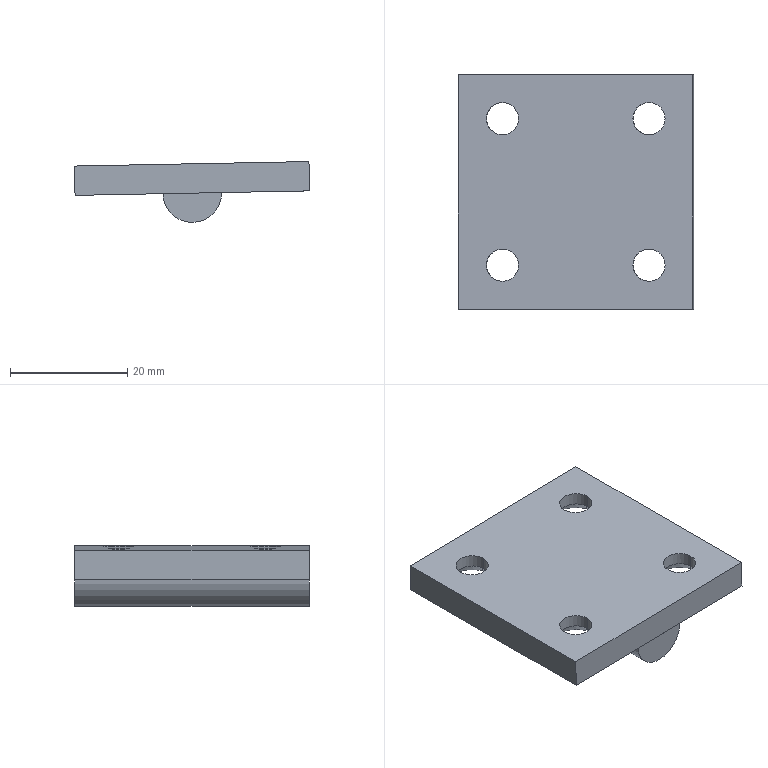Component | SolidWorks | 40X40AluminumAlloyHinge-4 | 2 solids | 27 faces | box 40.09 x 40 x 10.38 mm | volume 8718 mm3 | cylinder 10 | plane 9 | cone 8 | commonest cylinder face diameters 5.5 x8 10 x2 | material A3 Steel
build123d program:
from build123d import *

# Parameters (mm, degrees)
SKETCH1_W                                  = 40
SKETCH1_H                                  = 40
BOSS_EXTRUDE1_DEPTH                        = 5
BOSS_EXTRUDE2_DEPTH                        = 40
HOLE_SIZE_ACCORDING_TO_TYPE_1_OF_S_2_COUNT = 2
HOLE_SIZE_ACCORDING_TO_TYPE_1_OF_S_2_PITCH = 25
HOLE_SIZE_ACCORDING_TO_TYPE_1_OF_S_3_COUNT = 2
HOLE_SIZE_ACCORDING_TO_TYPE_1_OF_S_3_PITCH = 25
HOLE_SIZE_ACCORDING_TO_TYPE_1_OF_S_4_COUNT = 2
HOLE_SIZE_ACCORDING_TO_TYPE_1_OF_S_4_PITCH = 35.355


with BuildPart() as part:
    # Sketch1 → Boss-Extrude1 (new body)
    with BuildSketch(Plane.XY):
        Rectangle(SKETCH1_W, SKETCH1_H)
    extrude(amount=BOSS_EXTRUDE1_DEPTH)

    # Sketch5 → Hole Size _According to_ Type 1 of Slott (revolve, cut)
    with BuildSketch(Plane(origin=(-12.5, 12.5, 5), x_dir=(0, -1, 0), z_dir=(1, 0, 0))):
        Polygon((0, 0), (0, 5), (2.75, 5), (2.75, 2.85), (5.6, 0), align=None)
    hole_size_according_to_type_1_of_slott = revolve(axis=Axis((-12.5, 12.5, 11.35), (0, 0, -1)), mode=Mode.SUBTRACT)

    # Hole Size _According to_ Type 1 of S 2: Hole Size _According to_ Type 1 of Slott ×2
    with Locations(*[(0, -i * HOLE_SIZE_ACCORDING_TO_TYPE_1_OF_S_2_PITCH, 0) for i in range(1, HOLE_SIZE_ACCORDING_TO_TYPE_1_OF_S_2_COUNT)]):
        add(hole_size_according_to_type_1_of_slott, mode=Mode.SUBTRACT)

    # Hole Size _According to_ Type 1 of S 3: Hole Size _According to_ Type 1 of Slott ×2
    with Locations(*[(i * HOLE_SIZE_ACCORDING_TO_TYPE_1_OF_S_3_PITCH, 0, 0) for i in range(1, HOLE_SIZE_ACCORDING_TO_TYPE_1_OF_S_3_COUNT)]):
        add(hole_size_according_to_type_1_of_slott, mode=Mode.SUBTRACT)

    # Hole Size _According to_ Type 1 of S 4: Hole Size _According to_ Type 1 of Slott ×2
    with Locations(*[Vector(0.7071, -0.7071, 0) * (i * HOLE_SIZE_ACCORDING_TO_TYPE_1_OF_S_4_PITCH) for i in range(1, HOLE_SIZE_ACCORDING_TO_TYPE_1_OF_S_4_COUNT)]):
        add(hole_size_according_to_type_1_of_slott, mode=Mode.SUBTRACT)


with BuildPart() as body_2:
    # Sketch2 → Boss-Extrude2 (new body)
    with BuildSketch(Plane(origin=(0, 20, 0), x_dir=(1, 0, 0), z_dir=(0, 1, 0))):
        with BuildLine():
            Line((-5, -5), (5, -5))
            ThreePointArc((5, -5), (0, -10), (-5, -5))
        make_face()
    extrude(amount=-BOSS_EXTRUDE2_DEPTH)


solid = Compound([part.part, body_2.part])

# Placed as in the assembly
solid = solid.moved(Location((-505.846, -2233.022, 1470.376), (-180, 1.091, 0)))
STEP:
#1=COLOUR_RGB('',0.7922,0.8196,0.9333);
#2=FILL_AREA_STYLE_COLOUR('',#1);
#3=FILL_AREA_STYLE('',(#2));
#4=SURFACE_STYLE_FILL_AREA(#3);
#5=SURFACE_SIDE_STYLE('',(#4));
#6=SURFACE_STYLE_USAGE(.BOTH.,#5);
#7=PRESENTATION_STYLE_ASSIGNMENT((#6));
#8=CARTESIAN_POINT('',(-19.908,-87.127,57.495));
#9=VERTEX_POINT('',#8);
#10=CARTESIAN_POINT('',(-20.108,-87.127,57.688));
#11=VERTEX_POINT('',#10);
#12=CARTESIAN_POINT('',(-19.911,-87.127,57.692));
#13=DIRECTION('',(-0.,1.,-0.));
#14=DIRECTION('',(0.01904,0.,-0.9998));
#15=AXIS2_PLACEMENT_3D('',#12,#13,#14);
#16=CIRCLE('',#15,0.1969);
#17=EDGE_CURVE('',#9,#11,#16,.T.);
#18=ORIENTED_EDGE('',*,*,#17,.F.);
#19=CARTESIAN_POINT('',(-19.908,-88.702,57.495));
#20=VERTEX_POINT('',#19);
#21=CARTESIAN_POINT('',(-19.908,-86.687,57.495));
#22=DIRECTION('',(0.,-1.,0.));
#23=VECTOR('',#22,39.37);
#24=LINE('',#21,#23);
#25=EDGE_CURVE('',#9,#20,#24,.T.);
#26=ORIENTED_EDGE('',*,*,#25,.T.);
#27=CARTESIAN_POINT('',(-20.108,-88.702,57.688));
#28=VERTEX_POINT('',#27);
#29=CARTESIAN_POINT('',(-19.911,-88.702,57.692));
#30=DIRECTION('',(0.,-1.,0.));
#31=DIRECTION('',(0.01904,0.,-0.9998));
#32=AXIS2_PLACEMENT_3D('',#29,#30,#31);
#33=CIRCLE('',#32,0.1969);
#34=EDGE_CURVE('',#28,#20,#33,.T.);
#35=ORIENTED_EDGE('',*,*,#34,.F.);
#36=CARTESIAN_POINT('',(-20.108,-86.687,57.688));
#37=DIRECTION('',(0.,-1.,0.));
#38=VECTOR('',#37,39.37);
#39=LINE('',#36,#38);
#40=EDGE_CURVE('',#11,#28,#39,.T.);
#41=ORIENTED_EDGE('',*,*,#40,.F.);
#42=EDGE_LOOP('',(#18,#26,#35,#41));
#43=FACE_OUTER_BOUND('',#42,.T.);
#44=CARTESIAN_POINT('',(-19.911,-86.687,57.692));
#45=DIRECTION('',(0.,-1.,0.));
#46=DIRECTION('',(0.01904,0.,-0.9998));
#47=AXIS2_PLACEMENT_3D('',#44,#45,#46);
#48=CYLINDRICAL_SURFACE('',#47,0.1969);
#49=ADVANCED_FACE('',(#43),#48,.T.);
#50=ORIENTED_EDGE('',*,*,#25,.F.);
#51=CARTESIAN_POINT('',(-19.715,-87.127,57.696));
#52=VERTEX_POINT('',#51);
#53=CARTESIAN_POINT('',(-19.911,-87.127,57.692));
#54=DIRECTION('',(-0.,1.,-0.));
#55=DIRECTION('',(0.01904,0.,-0.9998));
#56=AXIS2_PLACEMENT_3D('',#53,#54,#55);
#57=CIRCLE('',#56,0.1969);
#58=EDGE_CURVE('',#52,#9,#57,.T.);
#59=ORIENTED_EDGE('',*,*,#58,.F.);
#60=CARTESIAN_POINT('',(-19.715,-88.702,57.696));
#61=VERTEX_POINT('',#60);
#62=CARTESIAN_POINT('',(-19.715,-86.687,57.696));
#63=DIRECTION('',(0.,-1.,0.));
#64=VECTOR('',#63,39.37);
#65=LINE('',#62,#64);
#66=EDGE_CURVE('',#52,#61,#65,.T.);
#67=ORIENTED_EDGE('',*,*,#66,.T.);
#68=CARTESIAN_POINT('',(-19.911,-88.702,57.692));
#69=DIRECTION('',(0.,-1.,0.));
#70=DIRECTION('',(0.01904,0.,-0.9998));
#71=AXIS2_PLACEMENT_3D('',#68,#69,#70);
#72=CIRCLE('',#71,0.1969);
#73=EDGE_CURVE('',#20,#61,#72,.T.);
#74=ORIENTED_EDGE('',*,*,#73,.F.);
#75=EDGE_LOOP('',(#50,#59,#67,#74));
#76=FACE_OUTER_BOUND('',#75,.T.);
#77=CARTESIAN_POINT('',(-19.911,-86.687,57.692));
#78=DIRECTION('',(0.,-1.,0.));
#79=DIRECTION('',(0.01904,0.,-0.9998));
#80=AXIS2_PLACEMENT_3D('',#77,#78,#79);
#81=CYLINDRICAL_SURFACE('',#80,0.1969);
#82=ADVANCED_FACE('',(#76),#81,.T.);
#83=CARTESIAN_POINT('',(-20.108,-87.127,57.688));
#84=DIRECTION('',(0.9998,0.,0.01904));
#85=VECTOR('',#84,39.37);
#86=LINE('',#83,#85);
#87=EDGE_CURVE('',#11,#52,#86,.T.);
#88=ORIENTED_EDGE('',*,*,#87,.F.);
#89=ORIENTED_EDGE('',*,*,#40,.T.);
#90=CARTESIAN_POINT('',(-20.108,-88.702,57.688));
#91=DIRECTION('',(-0.9998,-0.,-0.01904));
#92=VECTOR('',#91,39.37);
#93=LINE('',#90,#92);
#94=EDGE_CURVE('',#61,#28,#93,.T.);
#95=ORIENTED_EDGE('',*,*,#94,.F.);
#96=ORIENTED_EDGE('',*,*,#66,.F.);
#97=EDGE_LOOP('',(#88,#89,#95,#96));
#98=FACE_OUTER_BOUND('',#97,.T.);
#99=CARTESIAN_POINT('',(-20.108,-86.687,57.688));
#100=DIRECTION('',(-0.01904,0.,0.9998));
#101=DIRECTION('',(-0.9998,-0.,-0.01904));
#102=AXIS2_PLACEMENT_3D('',#99,#100,#101);
#103=PLANE('',#102);
#104=ADVANCED_FACE('',(#98),#103,.T.);
#105=ORIENTED_EDGE('',*,*,#34,.T.);
#106=ORIENTED_EDGE('',*,*,#73,.T.);
#107=ORIENTED_EDGE('',*,*,#94,.T.);
#108=EDGE_LOOP('',(#105,#106,#107));
#109=FACE_OUTER_BOUND('',#108,.T.);
#110=CARTESIAN_POINT('',(-19.911,-88.702,57.692));
#111=DIRECTION('',(0.,-1.,0.));
#112=DIRECTION('',(0.01904,-0.,-0.9998));
#113=AXIS2_PLACEMENT_3D('',#110,#111,#112);
#114=PLANE('',#113);
#115=ADVANCED_FACE('',(#109),#114,.T.);
#116=ORIENTED_EDGE('',*,*,#58,.T.);
#117=ORIENTED_EDGE('',*,*,#17,.T.);
#118=ORIENTED_EDGE('',*,*,#87,.T.);
#119=EDGE_LOOP('',(#116,#117,#118));
#120=FACE_OUTER_BOUND('',#119,.T.);
#121=CARTESIAN_POINT('',(-20.699,-87.127,57.677));
#122=DIRECTION('',(0.,-1.,0.));
#123=DIRECTION('',(0.01904,-0.,-0.9998));
#124=AXIS2_PLACEMENT_3D('',#121,#122,#123);
#125=PLANE('',#124);
#126=ADVANCED_FACE('',(#120),#125,.F.);
#127=CLOSED_SHELL('',(#49,#82,#104,#115,#126));
#128=MANIFOLD_SOLID_BREP('',#127);
#129=STYLED_ITEM('',(#7),#128);
#130=(LENGTH_UNIT()NAMED_UNIT(*)SI_UNIT($,.METRE.));
#131=LENGTH_MEASURE_WITH_UNIT(LENGTH_MEASURE(0.0254),#130);
#132=DIMENSIONAL_EXPONENTS(1.,0.,0.,0.,0.,0.,0.);
#133=(CONVERSION_BASED_UNIT('',#131)LENGTH_UNIT()NAMED_UNIT(#132));
#134=UNCERTAINTY_MEASURE_WITH_UNIT(LENGTH_MEASURE(0.00001),#133,'','');
#135=(NAMED_UNIT(*)PLANE_ANGLE_UNIT()SI_UNIT($,.RADIAN.));
#136=(NAMED_UNIT(*)SI_UNIT($,.STERADIAN.)SOLID_ANGLE_UNIT());
#137=(GEOMETRIC_REPRESENTATION_CONTEXT(3)GLOBAL_UNCERTAINTY_ASSIGNED_CONTEXT((#134))GLOBAL_UNIT_ASSIGNED_CONTEXT((#133,#135,#136))REPRESENTATION_CONTEXT('',''));
#138=MECHANICAL_DESIGN_GEOMETRIC_PRESENTATION_REPRESENTATION('',(#129),#137);
#139=COLOUR_RGB('',0.7922,0.8196,0.9333);
#140=FILL_AREA_STYLE_COLOUR('',#139);
#141=FILL_AREA_STYLE('',(#140));
#142=SURFACE_STYLE_FILL_AREA(#141);
#143=SURFACE_SIDE_STYLE('',(#142));
#144=SURFACE_STYLE_USAGE(.BOTH.,#143);
#145=PRESENTATION_STYLE_ASSIGNMENT((#144));
#146=CARTESIAN_POINT('',(-20.514,-88.406,57.793));
#147=VERTEX_POINT('',#146);
#148=CARTESIAN_POINT('',(-20.297,-88.406,57.797));
#149=VERTEX_POINT('',#148);
#150=CARTESIAN_POINT('',(-20.406,-88.406,57.795));
#151=DIRECTION('',(0.01904,-0.,-0.9998));
#152=DIRECTION('',(0.9998,0.,0.01904));
#153=AXIS2_PLACEMENT_3D('',#150,#151,#152);
#154=CIRCLE('',#153,0.1083);
#155=EDGE_CURVE('',#147,#149,#154,.T.);
#156=ORIENTED_EDGE('',*,*,#155,.F.);
#157=CARTESIAN_POINT('',(-20.624,-88.406,57.678));
#158=VERTEX_POINT('',#157);
#159=CARTESIAN_POINT('',(-20.624,-88.406,57.678));
#160=DIRECTION('',(-0.6935,-0.,-0.7204));
#161=VECTOR('',#160,39.37);
#162=LINE('',#159,#161);
#163=EDGE_CURVE('',#147,#158,#162,.T.);
#164=ORIENTED_EDGE('',*,*,#163,.T.);
#165=CARTESIAN_POINT('',(-20.183,-88.406,57.687));
#166=VERTEX_POINT('',#165);
#167=CARTESIAN_POINT('',(-20.404,-88.406,57.683));
#168=DIRECTION('',(0.01904,-0.,-0.9998));
#169=DIRECTION('',(0.9998,0.,0.01904));
#170=AXIS2_PLACEMENT_3D('',#167,#168,#169);
#171=CIRCLE('',#170,0.2205);
#172=EDGE_CURVE('',#158,#166,#171,.T.);
#173=ORIENTED_EDGE('',*,*,#172,.T.);
#174=CARTESIAN_POINT('',(-20.183,-88.406,57.687));
#175=DIRECTION('',(0.7204,0.,-0.6935));
#176=VECTOR('',#175,39.37);
#177=LINE('',#174,#176);
#178=EDGE_CURVE('',#149,#166,#177,.T.);
#179=ORIENTED_EDGE('',*,*,#178,.F.);
#180=EDGE_LOOP('',(#156,#164,#173,#179));
#181=FACE_OUTER_BOUND('',#180,.T.);
#182=CARTESIAN_POINT('',(-20.404,-88.406,57.683));
#183=DIRECTION('',(0.01904,-0.,-0.9998));
#184=DIRECTION('',(0.9998,0.,0.01904));
#185=AXIS2_PLACEMENT_3D('',#182,#183,#184);
#186=CONICAL_SURFACE('',#185,0.2205,0.7854);
#187=ADVANCED_FACE('',(#181),#186,.F.);
#188=CARTESIAN_POINT('',(-20.515,-88.406,57.877));
#189=VERTEX_POINT('',#188);
#190=CARTESIAN_POINT('',(-20.299,-88.406,57.881));
#191=VERTEX_POINT('',#190);
#192=CARTESIAN_POINT('',(-20.407,-88.406,57.879));
#193=DIRECTION('',(0.01904,-0.,-0.9998));
#194=DIRECTION('',(0.9998,0.,0.01904));
#195=AXIS2_PLACEMENT_3D('',#192,#193,#194);
#196=CIRCLE('',#195,0.1083);
#197=EDGE_CURVE('',#189,#191,#196,.T.);
#198=ORIENTED_EDGE('',*,*,#197,.F.);
#199=CARTESIAN_POINT('',(-20.512,-88.406,57.681));
#200=DIRECTION('',(0.01904,-0.,-0.9998));
#201=VECTOR('',#200,39.37);
#202=LINE('',#199,#201);
#203=EDGE_CURVE('',#189,#147,#202,.T.);
#204=ORIENTED_EDGE('',*,*,#203,.T.);
#205=ORIENTED_EDGE('',*,*,#155,.T.);
#206=CARTESIAN_POINT('',(-20.295,-88.406,57.685));
#207=DIRECTION('',(0.01904,-0.,-0.9998));
#208=VECTOR('',#207,39.37);
#209=LINE('',#206,#208);
#210=EDGE_CURVE('',#191,#149,#209,.T.);
#211=ORIENTED_EDGE('',*,*,#210,.F.);
#212=EDGE_LOOP('',(#198,#204,#205,#211));
#213=FACE_OUTER_BOUND('',#212,.T.);
#214=CARTESIAN_POINT('',(-20.404,-88.406,57.683));
#215=DIRECTION('',(0.01904,-0.,-0.9998));
#216=DIRECTION('',(0.9998,0.,0.01904));
#217=AXIS2_PLACEMENT_3D('',#214,#215,#216);
#218=CYLINDRICAL_SURFACE('',#217,0.1083);
#219=ADVANCED_FACE('',(#213),#218,.F.);
#220=CARTESIAN_POINT('',(-20.514,-87.422,57.793));
#221=VERTEX_POINT('',#220);
#222=CARTESIAN_POINT('',(-20.297,-87.422,57.797));
#223=VERTEX_POINT('',#222);
#224=CARTESIAN_POINT('',(-20.406,-87.422,57.795));
#225=DIRECTION('',(0.01904,-0.,-0.9998));
#226=DIRECTION('',(0.9998,0.,0.01904));
#227=AXIS2_PLACEMENT_3D('',#224,#225,#226);
#228=CIRCLE('',#227,0.1083);
#229=EDGE_CURVE('',#221,#223,#228,.T.);
#230=ORIENTED_EDGE('',*,*,#229,.F.);
#231=CARTESIAN_POINT('',(-20.624,-87.422,57.678));
#232=VERTEX_POINT('',#231);
#233=CARTESIAN_POINT('',(-20.624,-87.422,57.678));
#234=DIRECTION('',(-0.6935,-0.,-0.7204));
#235=VECTOR('',#234,39.37);
#236=LINE('',#233,#235);
#237=EDGE_CURVE('',#221,#232,#236,.T.);
#238=ORIENTED_EDGE('',*,*,#237,.T.);
#239=CARTESIAN_POINT('',(-20.183,-87.422,57.687));
#240=VERTEX_POINT('',#239);
#241=CARTESIAN_POINT('',(-20.404,-87.422,57.683));
#242=DIRECTION('',(0.01904,-0.,-0.9998));
#243=DIRECTION('',(0.9998,0.,0.01904));
#244=AXIS2_PLACEMENT_3D('',#241,#242,#243);
#245=CIRCLE('',#244,0.2205);
#246=EDGE_CURVE('',#232,#240,#245,.T.);
#247=ORIENTED_EDGE('',*,*,#246,.T.);
#248=CARTESIAN_POINT('',(-20.183,-87.422,57.687));
#249=DIRECTION('',(0.7204,0.,-0.6935));
#250=VECTOR('',#249,39.37);
#251=LINE('',#248,#250);
#252=EDGE_CURVE('',#223,#240,#251,.T.);
#253=ORIENTED_EDGE('',*,*,#252,.F.);
#254=EDGE_LOOP('',(#230,#238,#247,#253));
#255=FACE_OUTER_BOUND('',#254,.T.);
#256=CARTESIAN_POINT('',(-20.404,-87.422,57.683));
#257=DIRECTION('',(0.01904,-0.,-0.9998));
#258=DIRECTION('',(0.9998,0.,0.01904));
#259=AXIS2_PLACEMENT_3D('',#256,#257,#258);
#260=CONICAL_SURFACE('',#259,0.2205,0.7854);
#261=ADVANCED_FACE('',(#255),#260,.F.);
#262=CARTESIAN_POINT('',(-20.515,-87.422,57.877));
#263=VERTEX_POINT('',#262);
#264=CARTESIAN_POINT('',(-20.299,-87.422,57.881));
#265=VERTEX_POINT('',#264);
#266=CARTESIAN_POINT('',(-20.407,-87.422,57.879));
#267=DIRECTION('',(0.01904,-0.,-0.9998));
#268=DIRECTION('',(0.9998,0.,0.01904));
#269=AXIS2_PLACEMENT_3D('',#266,#267,#268);
#270=CIRCLE('',#269,0.1083);
#271=EDGE_CURVE('',#263,#265,#270,.T.);
#272=ORIENTED_EDGE('',*,*,#271,.F.);
#273=CARTESIAN_POINT('',(-20.512,-87.422,57.681));
#274=DIRECTION('',(0.01904,-0.,-0.9998));
#275=VECTOR('',#274,39.37);
#276=LINE('',#273,#275);
#277=EDGE_CURVE('',#263,#221,#276,.T.);
#278=ORIENTED_EDGE('',*,*,#277,.T.);
#279=ORIENTED_EDGE('',*,*,#229,.T.);
#280=CARTESIAN_POINT('',(-20.295,-87.422,57.685));
#281=DIRECTION('',(0.01904,-0.,-0.9998));
#282=VECTOR('',#281,39.37);
#283=LINE('',#280,#282);
#284=EDGE_CURVE('',#265,#223,#283,.T.);
#285=ORIENTED_EDGE('',*,*,#284,.F.);
#286=EDGE_LOOP('',(#272,#278,#279,#285));
#287=FACE_OUTER_BOUND('',#286,.T.);
#288=CARTESIAN_POINT('',(-20.404,-87.422,57.683));
#289=DIRECTION('',(0.01904,-0.,-0.9998));
#290=DIRECTION('',(0.9998,0.,0.01904));
#291=AXIS2_PLACEMENT_3D('',#288,#289,#290);
#292=CYLINDRICAL_SURFACE('',#291,0.1083);
#293=ADVANCED_FACE('',(#287),#292,.F.);
#294=CARTESIAN_POINT('',(-19.53,-88.406,57.811));
#295=VERTEX_POINT('',#294);
#296=CARTESIAN_POINT('',(-19.313,-88.406,57.816));
#297=VERTEX_POINT('',#296);
#298=CARTESIAN_POINT('',(-19.422,-88.406,57.814));
#299=DIRECTION('',(0.01904,-0.,-0.9998));
#300=DIRECTION('',(0.9998,0.,0.01904));
#301=AXIS2_PLACEMENT_3D('',#298,#299,#300);
#302=CIRCLE('',#301,0.1083);
#303=EDGE_CURVE('',#295,#297,#302,.T.);
#304=ORIENTED_EDGE('',*,*,#303,.F.);
#305=CARTESIAN_POINT('',(-19.64,-88.406,57.697));
#306=VERTEX_POINT('',#305);
#307=CARTESIAN_POINT('',(-19.64,-88.406,57.697));
#308=DIRECTION('',(-0.6935,-0.,-0.7204));
#309=VECTOR('',#308,39.37);
#310=LINE('',#307,#309);
#311=EDGE_CURVE('',#295,#306,#310,.T.);
#312=ORIENTED_EDGE('',*,*,#311,.T.);
#313=CARTESIAN_POINT('',(-19.199,-88.406,57.706));
#314=VERTEX_POINT('',#313);
#315=CARTESIAN_POINT('',(-19.419,-88.406,57.701));
#316=DIRECTION('',(0.01904,-0.,-0.9998));
#317=DIRECTION('',(0.9998,0.,0.01904));
#318=AXIS2_PLACEMENT_3D('',#315,#316,#317);
#319=CIRCLE('',#318,0.2205);
#320=EDGE_CURVE('',#306,#314,#319,.T.);
#321=ORIENTED_EDGE('',*,*,#320,.T.);
#322=CARTESIAN_POINT('',(-19.199,-88.406,57.706));
#323=DIRECTION('',(0.7204,0.,-0.6935));
#324=VECTOR('',#323,39.37);
#325=LINE('',#322,#324);
#326=EDGE_CURVE('',#297,#314,#325,.T.);
#327=ORIENTED_EDGE('',*,*,#326,.F.);
#328=EDGE_LOOP('',(#304,#312,#321,#327));
#329=FACE_OUTER_BOUND('',#328,.T.);
#330=CARTESIAN_POINT('',(-19.419,-88.406,57.701));
#331=DIRECTION('',(0.01904,-0.,-0.9998));
#332=DIRECTION('',(0.9998,0.,0.01904));
#333=AXIS2_PLACEMENT_3D('',#330,#331,#332);
#334=CONICAL_SURFACE('',#333,0.2205,0.7854);
#335=ADVANCED_FACE('',(#329),#334,.F.);
#336=CARTESIAN_POINT('',(-19.531,-88.406,57.896));
#337=VERTEX_POINT('',#336);
#338=CARTESIAN_POINT('',(-19.315,-88.406,57.9));
#339=VERTEX_POINT('',#338);
#340=CARTESIAN_POINT('',(-19.423,-88.406,57.898));
#341=DIRECTION('',(0.01904,-0.,-0.9998));
#342=DIRECTION('',(0.9998,0.,0.01904));
#343=AXIS2_PLACEMENT_3D('',#340,#341,#342);
#344=CIRCLE('',#343,0.1083);
#345=EDGE_CURVE('',#337,#339,#344,.T.);
#346=ORIENTED_EDGE('',*,*,#345,.F.);
#347=CARTESIAN_POINT('',(-19.528,-88.406,57.699));
#348=DIRECTION('',(0.01904,-0.,-0.9998));
#349=VECTOR('',#348,39.37);
#350=LINE('',#347,#349);
#351=EDGE_CURVE('',#337,#295,#350,.T.);
#352=ORIENTED_EDGE('',*,*,#351,.T.);
#353=ORIENTED_EDGE('',*,*,#303,.T.);
#354=CARTESIAN_POINT('',(-19.311,-88.406,57.703));
#355=DIRECTION('',(0.01904,-0.,-0.9998));
#356=VECTOR('',#355,39.37);
#357=LINE('',#354,#356);
#358=EDGE_CURVE('',#339,#297,#357,.T.);
#359=ORIENTED_EDGE('',*,*,#358,.F.);
#360=EDGE_LOOP('',(#346,#352,#353,#359));
#361=FACE_OUTER_BOUND('',#360,.T.);
#362=CARTESIAN_POINT('',(-19.419,-88.406,57.701));
#363=DIRECTION('',(0.01904,-0.,-0.9998));
#364=DIRECTION('',(0.9998,0.,0.01904));
#365=AXIS2_PLACEMENT_3D('',#362,#363,#364);
#366=CYLINDRICAL_SURFACE('',#365,0.1083);
#367=ADVANCED_FACE('',(#361),#366,.F.);
#368=CARTESIAN_POINT('',(-19.53,-87.422,57.811));
#369=VERTEX_POINT('',#368);
#370=CARTESIAN_POINT('',(-19.313,-87.422,57.816));
#371=VERTEX_POINT('',#370);
#372=CARTESIAN_POINT('',(-19.422,-87.422,57.814));
#373=DIRECTION('',(0.01904,-0.,-0.9998));
#374=DIRECTION('',(0.9998,0.,0.01904));
#375=AXIS2_PLACEMENT_3D('',#372,#373,#374);
#376=CIRCLE('',#375,0.1083);
#377=EDGE_CURVE('',#369,#371,#376,.T.);
#378=ORIENTED_EDGE('',*,*,#377,.F.);
#379=CARTESIAN_POINT('',(-19.64,-87.422,57.697));
#380=VERTEX_POINT('',#379);
#381=CARTESIAN_POINT('',(-19.64,-87.422,57.697));
#382=DIRECTION('',(-0.6935,-0.,-0.7204));
#383=VECTOR('',#382,39.37);
#384=LINE('',#381,#383);
#385=EDGE_CURVE('',#369,#380,#384,.T.);
#386=ORIENTED_EDGE('',*,*,#385,.T.);
#387=CARTESIAN_POINT('',(-19.199,-87.422,57.706));
#388=VERTEX_POINT('',#387);
#389=CARTESIAN_POINT('',(-19.419,-87.422,57.701));
#390=DIRECTION('',(0.01904,-0.,-0.9998));
#391=DIRECTION('',(0.9998,0.,0.01904));
#392=AXIS2_PLACEMENT_3D('',#389,#390,#391);
#393=CIRCLE('',#392,0.2205);
#394=EDGE_CURVE('',#380,#388,#393,.T.);
#395=ORIENTED_EDGE('',*,*,#394,.T.);
#396=CARTESIAN_POINT('',(-19.199,-87.422,57.706));
#397=DIRECTION('',(0.7204,0.,-0.6935));
#398=VECTOR('',#397,39.37);
#399=LINE('',#396,#398);
#400=EDGE_CURVE('',#371,#388,#399,.T.);
#401=ORIENTED_EDGE('',*,*,#400,.F.);
#402=EDGE_LOOP('',(#378,#386,#395,#401));
#403=FACE_OUTER_BOUND('',#402,.T.);
#404=CARTESIAN_POINT('',(-19.419,-87.422,57.701));
#405=DIRECTION('',(0.01904,-0.,-0.9998));
#406=DIRECTION('',(0.9998,0.,0.01904));
#407=AXIS2_PLACEMENT_3D('',#404,#405,#406);
#408=CONICAL_SURFACE('',#407,0.2205,0.7854);
#409=ADVANCED_FACE('',(#403),#408,.F.);
#410=CARTESIAN_POINT('',(-19.531,-87.422,57.896));
#411=VERTEX_POINT('',#410);
#412=CARTESIAN_POINT('',(-19.315,-87.422,57.9));
#413=VERTEX_POINT('',#412);
#414=CARTESIAN_POINT('',(-19.423,-87.422,57.898));
#415=DIRECTION('',(0.01904,-0.,-0.9998));
#416=DIRECTION('',(0.9998,0.,0.01904));
#417=AXIS2_PLACEMENT_3D('',#414,#415,#416);
#418=CIRCLE('',#417,0.1083);
#419=EDGE_CURVE('',#411,#413,#418,.T.);
#420=ORIENTED_EDGE('',*,*,#419,.F.);
#421=CARTESIAN_POINT('',(-19.528,-87.422,57.699));
#422=DIRECTION('',(0.01904,-0.,-0.9998));
#423=VECTOR('',#422,39.37);
#424=LINE('',#421,#423);
#425=EDGE_CURVE('',#411,#369,#424,.T.);
#426=ORIENTED_EDGE('',*,*,#425,.T.);
#427=ORIENTED_EDGE('',*,*,#377,.T.);
#428=CARTESIAN_POINT('',(-19.311,-87.422,57.703));
#429=DIRECTION('',(0.01904,-0.,-0.9998));
#430=VECTOR('',#429,39.37);
#431=LINE('',#428,#430);
#432=EDGE_CURVE('',#413,#371,#431,.T.);
#433=ORIENTED_EDGE('',*,*,#432,.F.);
#434=EDGE_LOOP('',(#420,#426,#427,#433));
#435=FACE_OUTER_BOUND('',#434,.T.);
#436=CARTESIAN_POINT('',(-19.419,-87.422,57.701));
#437=DIRECTION('',(0.01904,-0.,-0.9998));
#438=DIRECTION('',(0.9998,0.,0.01904));
#439=AXIS2_PLACEMENT_3D('',#436,#437,#438);
#440=CYLINDRICAL_SURFACE('',#439,0.1083);
#441=ADVANCED_FACE('',(#435),#440,.F.);
#442=CARTESIAN_POINT('',(-19.128,-87.127,57.904));
#443=VERTEX_POINT('',#442);
#444=CARTESIAN_POINT('',(-19.128,-88.702,57.904));
#445=VERTEX_POINT('',#444);
#446=CARTESIAN_POINT('',(-19.128,-87.127,57.904));
#447=DIRECTION('',(0.,-1.,0.));
#448=VECTOR('',#447,39.37);
#449=LINE('',#446,#448);
#450=EDGE_CURVE('',#443,#445,#449,.T.);
#451=ORIENTED_EDGE('',*,*,#450,.T.);
#452=CARTESIAN_POINT('',(-19.124,-88.702,57.707));
#453=VERTEX_POINT('',#452);
#454=CARTESIAN_POINT('',(-19.124,-88.702,57.707));
#455=DIRECTION('',(-0.01904,0.,0.9998));
#456=VECTOR('',#455,39.37);
#457=LINE('',#454,#456);
#458=EDGE_CURVE('',#453,#445,#457,.T.);
#459=ORIENTED_EDGE('',*,*,#458,.F.);
#460=CARTESIAN_POINT('',(-19.124,-87.127,57.707));
#461=VERTEX_POINT('',#460);
#462=CARTESIAN_POINT('',(-19.124,-87.127,57.707));
#463=DIRECTION('',(0.,-1.,0.));
#464=VECTOR('',#463,39.37);
#465=LINE('',#462,#464);
#466=EDGE_CURVE('',#461,#453,#465,.T.);
#467=ORIENTED_EDGE('',*,*,#466,.F.);
#468=CARTESIAN_POINT('',(-19.124,-87.127,57.707));
#469=DIRECTION('',(-0.01904,0.,0.9998));
#470=VECTOR('',#469,39.37);
#471=LINE('',#468,#470);
#472=EDGE_CURVE('',#461,#443,#471,.T.);
#473=ORIENTED_EDGE('',*,*,#472,.T.);
#474=EDGE_LOOP('',(#451,#459,#467,#473));
#475=FACE_OUTER_BOUND('',#474,.T.);
#476=CARTESIAN_POINT('',(-19.124,-87.127,57.707));
#477=DIRECTION('',(-0.9998,-0.,-0.01904));
#478=DIRECTION('',(0.01904,-0.,-0.9998));
#479=AXIS2_PLACEMENT_3D('',#476,#477,#478);
#480=PLANE('',#479);
#481=ADVANCED_FACE('',(#475),#480,.F.);
#482=CARTESIAN_POINT('',(-20.702,-88.702,57.874));
#483=VERTEX_POINT('',#482);
#484=CARTESIAN_POINT('',(-20.702,-88.702,57.874));
#485=DIRECTION('',(-0.9998,-0.,-0.01904));
#486=VECTOR('',#485,39.37);
#487=LINE('',#484,#486);
#488=EDGE_CURVE('',#445,#483,#487,.T.);
#489=ORIENTED_EDGE('',*,*,#488,.T.);
#490=CARTESIAN_POINT('',(-20.699,-88.702,57.677));
#491=VERTEX_POINT('',#490);
#492=CARTESIAN_POINT('',(-20.699,-88.702,57.677));
#493=DIRECTION('',(-0.01904,0.,0.9998));
#494=VECTOR('',#493,39.37);
#495=LINE('',#492,#494);
#496=EDGE_CURVE('',#491,#483,#495,.T.);
#497=ORIENTED_EDGE('',*,*,#496,.F.);
#498=CARTESIAN_POINT('',(-20.699,-88.702,57.677));
#499=DIRECTION('',(-0.9998,-0.,-0.01904));
#500=VECTOR('',#499,39.37);
#501=LINE('',#498,#500);
#502=EDGE_CURVE('',#453,#491,#501,.T.);
#503=ORIENTED_EDGE('',*,*,#502,.F.);
#504=ORIENTED_EDGE('',*,*,#458,.T.);
#505=EDGE_LOOP('',(#489,#497,#503,#504));
#506=FACE_OUTER_BOUND('',#505,.T.);
#507=CARTESIAN_POINT('',(-20.699,-88.702,57.677));
#508=DIRECTION('',(-0.,1.,-0.));
#509=DIRECTION('',(-0.01904,0.,0.9998));
#510=AXIS2_PLACEMENT_3D('',#507,#508,#509);
#511=PLANE('',#510);
#512=ADVANCED_FACE('',(#506),#511,.F.);
#513=CARTESIAN_POINT('',(-20.702,-87.127,57.874));
#514=VERTEX_POINT('',#513);
#515=CARTESIAN_POINT('',(-20.702,-87.127,57.874));
#516=DIRECTION('',(-0.,1.,-0.));
#517=VECTOR('',#516,39.37);
#518=LINE('',#515,#517);
#519=EDGE_CURVE('',#483,#514,#518,.T.);
#520=ORIENTED_EDGE('',*,*,#519,.T.);
#521=CARTESIAN_POINT('',(-20.699,-87.127,57.677));
#522=VERTEX_POINT('',#521);
#523=CARTESIAN_POINT('',(-20.699,-87.127,57.677));
#524=DIRECTION('',(-0.01904,0.,0.9998));
#525=VECTOR('',#524,39.37);
#526=LINE('',#523,#525);
#527=EDGE_CURVE('',#522,#514,#526,.T.);
#528=ORIENTED_EDGE('',*,*,#527,.F.);
#529=CARTESIAN_POINT('',(-20.699,-87.127,57.677));
#530=DIRECTION('',(-0.,1.,-0.));
#531=VECTOR('',#530,39.37);
#532=LINE('',#529,#531);
#533=EDGE_CURVE('',#491,#522,#532,.T.);
#534=ORIENTED_EDGE('',*,*,#533,.F.);
#535=ORIENTED_EDGE('',*,*,#496,.T.);
#536=EDGE_LOOP('',(#520,#528,#534,#535));
#537=FACE_OUTER_BOUND('',#536,.T.);
#538=CARTESIAN_POINT('',(-20.699,-87.127,57.677));
#539=DIRECTION('',(0.9998,0.,0.01904));
#540=DIRECTION('',(-0.01904,0.,0.9998));
#541=AXIS2_PLACEMENT_3D('',#538,#539,#540);
#542=PLANE('',#541);
#543=ADVANCED_FACE('',(#537),#542,.F.);
#544=CARTESIAN_POINT('',(-20.702,-87.127,57.874));
#545=DIRECTION('',(0.9998,0.,0.01904));
#546=VECTOR('',#545,39.37);
#547=LINE('',#544,#546);
#548=EDGE_CURVE('',#514,#443,#547,.T.);
#549=ORIENTED_EDGE('',*,*,#548,.T.);
#550=ORIENTED_EDGE('',*,*,#472,.F.);
#551=CARTESIAN_POINT('',(-20.699,-87.127,57.677));
#552=DIRECTION('',(0.9998,0.,0.01904));
#553=VECTOR('',#552,39.37);
#554=LINE('',#551,#553);
#555=EDGE_CURVE('',#522,#461,#554,.T.);
#556=ORIENTED_EDGE('',*,*,#555,.F.);
#557=ORIENTED_EDGE('',*,*,#527,.T.);
#558=EDGE_LOOP('',(#549,#550,#556,#557));
#559=FACE_OUTER_BOUND('',#558,.T.);
#560=CARTESIAN_POINT('',(-20.699,-87.127,57.677));
#561=DIRECTION('',(0.,-1.,0.));
#562=DIRECTION('',(0.01904,-0.,-0.9998));
#563=AXIS2_PLACEMENT_3D('',#560,#561,#562);
#564=PLANE('',#563);
#565=ADVANCED_FACE('',(#559),#564,.F.);
#566=CARTESIAN_POINT('',(-20.404,-88.406,57.683));
#567=DIRECTION('',(0.01904,-0.,-0.9998));
#568=DIRECTION('',(0.9998,0.,0.01904));
#569=AXIS2_PLACEMENT_3D('',#566,#567,#568);
#570=CIRCLE('',#569,0.2205);
#571=EDGE_CURVE('',#166,#158,#570,.T.);
#572=ORIENTED_EDGE('',*,*,#571,.F.);
#573=ORIENTED_EDGE('',*,*,#172,.F.);
#574=EDGE_LOOP('',(#572,#573));
#575=FACE_BOUND('',#574,.T.);
#576=CARTESIAN_POINT('',(-20.404,-87.422,57.683));
#577=DIRECTION('',(0.01904,-0.,-0.9998));
#578=DIRECTION('',(0.9998,0.,0.01904));
#579=AXIS2_PLACEMENT_3D('',#576,#577,#578);
#580=CIRCLE('',#579,0.2205);
#581=EDGE_CURVE('',#240,#232,#580,.T.);
#582=ORIENTED_EDGE('',*,*,#581,.F.);
#583=ORIENTED_EDGE('',*,*,#246,.F.);
#584=EDGE_LOOP('',(#582,#583));
#585=FACE_BOUND('',#584,.T.);
#586=CARTESIAN_POINT('',(-19.419,-88.406,57.701));
#587=DIRECTION('',(0.01904,-0.,-0.9998));
#588=DIRECTION('',(0.9998,0.,0.01904));
#589=AXIS2_PLACEMENT_3D('',#586,#587,#588);
#590=CIRCLE('',#589,0.2205);
#591=EDGE_CURVE('',#314,#306,#590,.T.);
#592=ORIENTED_EDGE('',*,*,#591,.F.);
#593=ORIENTED_EDGE('',*,*,#320,.F.);
#594=EDGE_LOOP('',(#592,#593));
#595=FACE_BOUND('',#594,.T.);
#596=CARTESIAN_POINT('',(-19.419,-87.422,57.701));
#597=DIRECTION('',(0.01904,-0.,-0.9998));
#598=DIRECTION('',(0.9998,0.,0.01904));
#599=AXIS2_PLACEMENT_3D('',#596,#597,#598);
#600=CIRCLE('',#599,0.2205);
#601=EDGE_CURVE('',#388,#380,#600,.T.);
#602=ORIENTED_EDGE('',*,*,#601,.F.);
#603=ORIENTED_EDGE('',*,*,#394,.F.);
#604=EDGE_LOOP('',(#602,#603));
#605=FACE_BOUND('',#604,.T.);
#606=ORIENTED_EDGE('',*,*,#466,.T.);
#607=ORIENTED_EDGE('',*,*,#502,.T.);
#608=ORIENTED_EDGE('',*,*,#533,.T.);
#609=ORIENTED_EDGE('',*,*,#555,.T.);
#610=EDGE_LOOP('',(#606,#607,#608,#609));
#611=FACE_OUTER_BOUND('',#610,.T.);
#612=CARTESIAN_POINT('',(-19.911,-87.914,57.692));
#613=DIRECTION('',(-0.01904,0.,0.9998));
#614=DIRECTION('',(-0.9998,-0.,-0.01904));
#615=AXIS2_PLACEMENT_3D('',#612,#613,#614);
#616=PLANE('',#615);
#617=ADVANCED_FACE('',(#575,#585,#595,#605,#611),#616,.F.);
#618=CARTESIAN_POINT('',(-20.407,-88.406,57.879));
#619=DIRECTION('',(0.01904,-0.,-0.9998));
#620=DIRECTION('',(0.9998,0.,0.01904));
#621=AXIS2_PLACEMENT_3D('',#618,#619,#620);
#622=CIRCLE('',#621,0.1083);
#623=EDGE_CURVE('',#191,#189,#622,.T.);
#624=ORIENTED_EDGE('',*,*,#623,.T.);
#625=ORIENTED_EDGE('',*,*,#197,.T.);
#626=EDGE_LOOP('',(#624,#625));
#627=FACE_BOUND('',#626,.T.);
#628=CARTESIAN_POINT('',(-20.407,-87.422,57.879));
#629=DIRECTION('',(0.01904,-0.,-0.9998));
#630=DIRECTION('',(0.9998,0.,0.01904));
#631=AXIS2_PLACEMENT_3D('',#628,#629,#630);
#632=CIRCLE('',#631,0.1083);
#633=EDGE_CURVE('',#265,#263,#632,.T.);
#634=ORIENTED_EDGE('',*,*,#633,.T.);
#635=ORIENTED_EDGE('',*,*,#271,.T.);
#636=EDGE_LOOP('',(#634,#635));
#637=FACE_BOUND('',#636,.T.);
#638=CARTESIAN_POINT('',(-19.423,-88.406,57.898));
#639=DIRECTION('',(0.01904,-0.,-0.9998));
#640=DIRECTION('',(0.9998,0.,0.01904));
#641=AXIS2_PLACEMENT_3D('',#638,#639,#640);
#642=CIRCLE('',#641,0.1083);
#643=EDGE_CURVE('',#339,#337,#642,.T.);
#644=ORIENTED_EDGE('',*,*,#643,.T.);
#645=ORIENTED_EDGE('',*,*,#345,.T.);
#646=EDGE_LOOP('',(#644,#645));
#647=FACE_BOUND('',#646,.T.);
#648=CARTESIAN_POINT('',(-19.423,-87.422,57.898));
#649=DIRECTION('',(0.01904,-0.,-0.9998));
#650=DIRECTION('',(0.9998,0.,0.01904));
#651=AXIS2_PLACEMENT_3D('',#648,#649,#650);
#652=CIRCLE('',#651,0.1083);
#653=EDGE_CURVE('',#413,#411,#652,.T.);
#654=ORIENTED_EDGE('',*,*,#653,.T.);
#655=ORIENTED_EDGE('',*,*,#419,.T.);
#656=EDGE_LOOP('',(#654,#655));
#657=FACE_BOUND('',#656,.T.);
#658=ORIENTED_EDGE('',*,*,#450,.F.);
#659=ORIENTED_EDGE('',*,*,#548,.F.);
#660=ORIENTED_EDGE('',*,*,#519,.F.);
#661=ORIENTED_EDGE('',*,*,#488,.F.);
#662=EDGE_LOOP('',(#658,#659,#660,#661));
#663=FACE_OUTER_BOUND('',#662,.T.);
#664=CARTESIAN_POINT('',(-19.915,-87.914,57.889));
#665=DIRECTION('',(-0.01904,0.,0.9998));
#666=DIRECTION('',(-0.9998,-0.,-0.01904));
#667=AXIS2_PLACEMENT_3D('',#664,#665,#666);
#668=PLANE('',#667);
#669=ADVANCED_FACE('',(#627,#637,#647,#657,#663),#668,.T.);
#670=ORIENTED_EDGE('',*,*,#425,.F.);
#671=ORIENTED_EDGE('',*,*,#653,.F.);
#672=ORIENTED_EDGE('',*,*,#432,.T.);
#673=CARTESIAN_POINT('',(-19.422,-87.422,57.814));
#674=DIRECTION('',(0.01904,-0.,-0.9998));
#675=DIRECTION('',(0.9998,0.,0.01904));
#676=AXIS2_PLACEMENT_3D('',#673,#674,#675);
#677=CIRCLE('',#676,0.1083);
#678=EDGE_CURVE('',#371,#369,#677,.T.);
#679=ORIENTED_EDGE('',*,*,#678,.T.);
#680=EDGE_LOOP('',(#670,#671,#672,#679));
#681=FACE_OUTER_BOUND('',#680,.T.);
#682=CARTESIAN_POINT('',(-19.419,-87.422,57.701));
#683=DIRECTION('',(0.01904,-0.,-0.9998));
#684=DIRECTION('',(0.9998,0.,0.01904));
#685=AXIS2_PLACEMENT_3D('',#682,#683,#684);
#686=CYLINDRICAL_SURFACE('',#685,0.1083);
#687=ADVANCED_FACE('',(#681),#686,.F.);
#688=ORIENTED_EDGE('',*,*,#385,.F.);
#689=ORIENTED_EDGE('',*,*,#678,.F.);
#690=ORIENTED_EDGE('',*,*,#400,.T.);
#691=ORIENTED_EDGE('',*,*,#601,.T.);
#692=EDGE_LOOP('',(#688,#689,#690,#691));
#693=FACE_OUTER_BOUND('',#692,.T.);
#694=CARTESIAN_POINT('',(-19.419,-87.422,57.701));
#695=DIRECTION('',(0.01904,-0.,-0.9998));
#696=DIRECTION('',(0.9998,0.,0.01904));
#697=AXIS2_PLACEMENT_3D('',#694,#695,#696);
#698=CONICAL_SURFACE('',#697,0.2205,0.7854);
#699=ADVANCED_FACE('',(#693),#698,.F.);
#700=ORIENTED_EDGE('',*,*,#351,.F.);
#701=ORIENTED_EDGE('',*,*,#643,.F.);
#702=ORIENTED_EDGE('',*,*,#358,.T.);
#703=CARTESIAN_POINT('',(-19.422,-88.406,57.814));
#704=DIRECTION('',(0.01904,-0.,-0.9998));
#705=DIRECTION('',(0.9998,0.,0.01904));
#706=AXIS2_PLACEMENT_3D('',#703,#704,#705);
#707=CIRCLE('',#706,0.1083);
#708=EDGE_CURVE('',#297,#295,#707,.T.);
#709=ORIENTED_EDGE('',*,*,#708,.T.);
#710=EDGE_LOOP('',(#700,#701,#702,#709));
#711=FACE_OUTER_BOUND('',#710,.T.);
#712=CARTESIAN_POINT('',(-19.419,-88.406,57.701));
#713=DIRECTION('',(0.01904,-0.,-0.9998));
#714=DIRECTION('',(0.9998,0.,0.01904));
#715=AXIS2_PLACEMENT_3D('',#712,#713,#714);
#716=CYLINDRICAL_SURFACE('',#715,0.1083);
#717=ADVANCED_FACE('',(#711),#716,.F.);
#718=ORIENTED_EDGE('',*,*,#311,.F.);
#719=ORIENTED_EDGE('',*,*,#708,.F.);
#720=ORIENTED_EDGE('',*,*,#326,.T.);
#721=ORIENTED_EDGE('',*,*,#591,.T.);
#722=EDGE_LOOP('',(#718,#719,#720,#721));
#723=FACE_OUTER_BOUND('',#722,.T.);
#724=CARTESIAN_POINT('',(-19.419,-88.406,57.701));
#725=DIRECTION('',(0.01904,-0.,-0.9998));
#726=DIRECTION('',(0.9998,0.,0.01904));
#727=AXIS2_PLACEMENT_3D('',#724,#725,#726);
#728=CONICAL_SURFACE('',#727,0.2205,0.7854);
#729=ADVANCED_FACE('',(#723),#728,.F.);
#730=ORIENTED_EDGE('',*,*,#277,.F.);
#731=ORIENTED_EDGE('',*,*,#633,.F.);
#732=ORIENTED_EDGE('',*,*,#284,.T.);
#733=CARTESIAN_POINT('',(-20.406,-87.422,57.795));
#734=DIRECTION('',(0.01904,-0.,-0.9998));
#735=DIRECTION('',(0.9998,0.,0.01904));
#736=AXIS2_PLACEMENT_3D('',#733,#734,#735);
#737=CIRCLE('',#736,0.1083);
#738=EDGE_CURVE('',#223,#221,#737,.T.);
#739=ORIENTED_EDGE('',*,*,#738,.T.);
#740=EDGE_LOOP('',(#730,#731,#732,#739));
#741=FACE_OUTER_BOUND('',#740,.T.);
#742=CARTESIAN_POINT('',(-20.404,-87.422,57.683));
#743=DIRECTION('',(0.01904,-0.,-0.9998));
#744=DIRECTION('',(0.9998,0.,0.01904));
#745=AXIS2_PLACEMENT_3D('',#742,#743,#744);
#746=CYLINDRICAL_SURFACE('',#745,0.1083);
#747=ADVANCED_FACE('',(#741),#746,.F.);
#748=ORIENTED_EDGE('',*,*,#237,.F.);
#749=ORIENTED_EDGE('',*,*,#738,.F.);
#750=ORIENTED_EDGE('',*,*,#252,.T.);
#751=ORIENTED_EDGE('',*,*,#581,.T.);
#752=EDGE_LOOP('',(#748,#749,#750,#751));
#753=FACE_OUTER_BOUND('',#752,.T.);
#754=CARTESIAN_POINT('',(-20.404,-87.422,57.683));
#755=DIRECTION('',(0.01904,-0.,-0.9998));
#756=DIRECTION('',(0.9998,0.,0.01904));
#757=AXIS2_PLACEMENT_3D('',#754,#755,#756);
#758=CONICAL_SURFACE('',#757,0.2205,0.7854);
#759=ADVANCED_FACE('',(#753),#758,.F.);
#760=ORIENTED_EDGE('',*,*,#203,.F.);
#761=ORIENTED_EDGE('',*,*,#623,.F.);
#762=ORIENTED_EDGE('',*,*,#210,.T.);
#763=CARTESIAN_POINT('',(-20.406,-88.406,57.795));
#764=DIRECTION('',(0.01904,-0.,-0.9998));
#765=DIRECTION('',(0.9998,0.,0.01904));
#766=AXIS2_PLACEMENT_3D('',#763,#764,#765);
#767=CIRCLE('',#766,0.1083);
#768=EDGE_CURVE('',#149,#147,#767,.T.);
#769=ORIENTED_EDGE('',*,*,#768,.T.);
#770=EDGE_LOOP('',(#760,#761,#762,#769));
#771=FACE_OUTER_BOUND('',#770,.T.);
#772=CARTESIAN_POINT('',(-20.404,-88.406,57.683));
#773=DIRECTION('',(0.01904,-0.,-0.9998));
#774=DIRECTION('',(0.9998,0.,0.01904));
#775=AXIS2_PLACEMENT_3D('',#772,#773,#774);
#776=CYLINDRICAL_SURFACE('',#775,0.1083);
#777=ADVANCED_FACE('',(#771),#776,.F.);
#778=ORIENTED_EDGE('',*,*,#163,.F.);
#779=ORIENTED_EDGE('',*,*,#768,.F.);
#780=ORIENTED_EDGE('',*,*,#178,.T.);
#781=ORIENTED_EDGE('',*,*,#571,.T.);
#782=EDGE_LOOP('',(#778,#779,#780,#781));
#783=FACE_OUTER_BOUND('',#782,.T.);
#784=CARTESIAN_POINT('',(-20.404,-88.406,57.683));
#785=DIRECTION('',(0.01904,-0.,-0.9998));
#786=DIRECTION('',(0.9998,0.,0.01904));
#787=AXIS2_PLACEMENT_3D('',#784,#785,#786);
#788=CONICAL_SURFACE('',#787,0.2205,0.7854);
#789=ADVANCED_FACE('',(#783),#788,.F.);
#790=CLOSED_SHELL('',(#187,#219,#261,#293,#335,#367,#409,#441,#481,#512,#543,#565,#617,#669,#687,#699,#717,#729,#747,#759,#777,#789));
#791=MANIFOLD_SOLID_BREP('',#790);
#792=STYLED_ITEM('',(#145),#791);
#793=PRESENTATION_LAYER_ASSIGNMENT('','',(#792));
#794=CARTESIAN_POINT('',(0.,0.,0.));
#795=DIRECTION('',(0.,0.,1.));
#796=DIRECTION('',(1.,0.,0.));
#797=AXIS2_PLACEMENT_3D('',#794,#795,#796);
#798=(LENGTH_UNIT()NAMED_UNIT(*)SI_UNIT($,.METRE.));
#799=LENGTH_MEASURE_WITH_UNIT(LENGTH_MEASURE(0.0254),#798);
#800=DIMENSIONAL_EXPONENTS(1.,0.,0.,0.,0.,0.,0.);
#801=(CONVERSION_BASED_UNIT('',#799)LENGTH_UNIT()NAMED_UNIT(#800));
#802=UNCERTAINTY_MEASURE_WITH_UNIT(LENGTH_MEASURE(0.00001),#801,'','');
#803=(NAMED_UNIT(*)PLANE_ANGLE_UNIT()SI_UNIT($,.RADIAN.));
#804=(NAMED_UNIT(*)SI_UNIT($,.STERADIAN.)SOLID_ANGLE_UNIT());
#805=(GEOMETRIC_REPRESENTATION_CONTEXT(3)GLOBAL_UNCERTAINTY_ASSIGNED_CONTEXT((#802))GLOBAL_UNIT_ASSIGNED_CONTEXT((#801,#803,#804))REPRESENTATION_CONTEXT('',''));
#806=ADVANCED_BREP_SHAPE_REPRESENTATION('',(#128,#791,#797),#805);
#807=PRESENTATION_LAYER_ASSIGNMENT('','',(#129));
#808=(LENGTH_UNIT()NAMED_UNIT(*)SI_UNIT($,.METRE.));
#809=LENGTH_MEASURE_WITH_UNIT(LENGTH_MEASURE(0.0254),#808);
#810=DIMENSIONAL_EXPONENTS(1.,0.,0.,0.,0.,0.,0.);
#811=(CONVERSION_BASED_UNIT('',#809)LENGTH_UNIT()NAMED_UNIT(#810));
#812=UNCERTAINTY_MEASURE_WITH_UNIT(LENGTH_MEASURE(0.00001),#811,'','');
#813=(NAMED_UNIT(*)PLANE_ANGLE_UNIT()SI_UNIT($,.RADIAN.));
#814=(NAMED_UNIT(*)SI_UNIT($,.STERADIAN.)SOLID_ANGLE_UNIT());
#815=(GEOMETRIC_REPRESENTATION_CONTEXT(3)GLOBAL_UNCERTAINTY_ASSIGNED_CONTEXT((#812))GLOBAL_UNIT_ASSIGNED_CONTEXT((#811,#813,#814))REPRESENTATION_CONTEXT('',''));
#816=MECHANICAL_DESIGN_GEOMETRIC_PRESENTATION_REPRESENTATION('',(#792),#815);